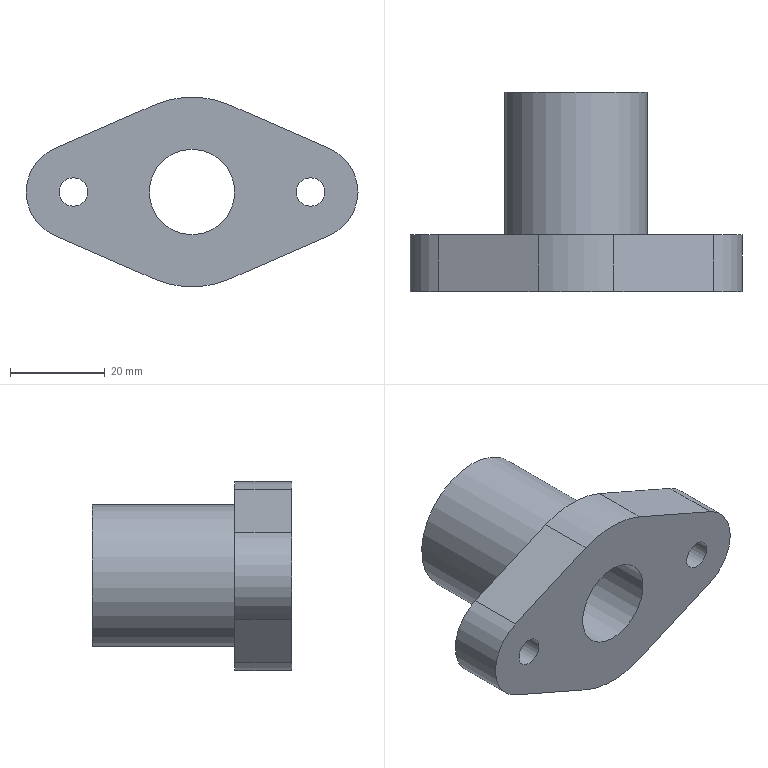Component | NX | GLAND | 1 solid | 15 faces | box 70 x 42 x 40 mm | volume 33070 mm3 | cylinder 8 | plane 7 | commonest cylinder face diameters 40 x2 20 x2 6 x2 30 x1 18 x1
STEP:
#1=CARTESIAN_POINT('',(0.,0.,0.));
#2=DIRECTION('',(0.,0.,1.));
#3=DIRECTION('',(1.,0.,0.));
#4=AXIS2_PLACEMENT_3D('',#1,#2,#3);
#5=CARTESIAN_POINT('',(-29.,-84.,-36.165));
#6=VERTEX_POINT('',#5);
#7=CARTESIAN_POINT('',(-8.,-84.,-45.33));
#8=VERTEX_POINT('',#7);
#9=CARTESIAN_POINT('',(-29.,-84.,-36.165));
#10=DIRECTION('',(0.9165,0.,-0.4));
#11=VECTOR('',#10,1.);
#12=LINE('',#9,#11);
#13=CARTESIAN_POINT('',(-29.,-72.,-36.165));
#14=DIRECTION('',(-0.4,0.,-0.9165));
#15=DIRECTION('',(0.9165,0.,-0.4));
#16=AXIS2_PLACEMENT_3D('',#13,#14,#15);
#17=PLANE('',#16);
#18=CARTESIAN_POINT('',(0.,12.));
#19=DIRECTION('',(1.,0.));
#20=VECTOR('',#19,1.);
#21=LINE('',#18,#20);
#22=(GEOMETRIC_REPRESENTATION_CONTEXT(2)PARAMETRIC_REPRESENTATION_CONTEXT()REPRESENTATION_CONTEXT('',''));
#23=DEFINITIONAL_REPRESENTATION('',(#21),#22);
#24=PCURVE('',#17,#23);
#25=CARTESIAN_POINT('',(0.,-84.,-27.));
#26=DIRECTION('',(0.,-1.,0.));
#27=DIRECTION('',(0.,0.,1.));
#28=AXIS2_PLACEMENT_3D('',#25,#26,#27);
#29=PLANE('',#28);
#30=CARTESIAN_POINT('',(-9.165,29.));
#31=DIRECTION('',(-0.4,-0.9165));
#32=VECTOR('',#31,1.);
#33=LINE('',#30,#32);
#34=(GEOMETRIC_REPRESENTATION_CONTEXT(2)PARAMETRIC_REPRESENTATION_CONTEXT()REPRESENTATION_CONTEXT('',''));
#35=DEFINITIONAL_REPRESENTATION('',(#33),#34);
#36=PCURVE('',#29,#35);
#37=SURFACE_CURVE('',#12,(#24,#36),.PCURVE_S1.);
#38=EDGE_CURVE('',#6,#8,#37,.T.);
#39=ORIENTED_EDGE('',*,*,#38,.F.);
#40=CARTESIAN_POINT('',(-29.,-72.,-36.165));
#41=VERTEX_POINT('',#40);
#42=CARTESIAN_POINT('',(-29.,-72.,-36.165));
#43=DIRECTION('',(0.,-1.,0.));
#44=VECTOR('',#43,1.);
#45=LINE('',#42,#44);
#46=CARTESIAN_POINT('',(0.,0.));
#47=DIRECTION('',(0.,1.));
#48=VECTOR('',#47,1.);
#49=LINE('',#46,#48);
#50=(GEOMETRIC_REPRESENTATION_CONTEXT(2)PARAMETRIC_REPRESENTATION_CONTEXT()REPRESENTATION_CONTEXT('',''));
#51=DEFINITIONAL_REPRESENTATION('',(#49),#50);
#52=PCURVE('',#17,#51);
#53=CARTESIAN_POINT('',(-25.,-72.,-27.));
#54=DIRECTION('',(0.,-1.,0.));
#55=DIRECTION('',(0.,0.,1.));
#56=AXIS2_PLACEMENT_3D('',#53,#54,#55);
#57=CYLINDRICAL_SURFACE('',#56,10.);
#58=CARTESIAN_POINT('',(2.73,0.));
#59=DIRECTION('',(0.,1.));
#60=VECTOR('',#59,1.);
#61=LINE('',#58,#60);
#62=(GEOMETRIC_REPRESENTATION_CONTEXT(2)PARAMETRIC_REPRESENTATION_CONTEXT()REPRESENTATION_CONTEXT('',''));
#63=DEFINITIONAL_REPRESENTATION('',(#61),#62);
#64=PCURVE('',#57,#63);
#65=SURFACE_CURVE('',#45,(#52,#64),.PCURVE_S1.);
#66=EDGE_CURVE('',#41,#6,#65,.T.);
#67=ORIENTED_EDGE('',*,*,#66,.F.);
#68=CARTESIAN_POINT('',(-8.,-72.,-45.33));
#69=VERTEX_POINT('',#68);
#70=CARTESIAN_POINT('',(-29.,-72.,-36.165));
#71=DIRECTION('',(0.9165,0.,-0.4));
#72=VECTOR('',#71,1.);
#73=LINE('',#70,#72);
#74=CARTESIAN_POINT('',(0.,0.));
#75=DIRECTION('',(1.,0.));
#76=VECTOR('',#75,1.);
#77=LINE('',#74,#76);
#78=(GEOMETRIC_REPRESENTATION_CONTEXT(2)PARAMETRIC_REPRESENTATION_CONTEXT()REPRESENTATION_CONTEXT('',''));
#79=DEFINITIONAL_REPRESENTATION('',(#77),#78);
#80=PCURVE('',#17,#79);
#81=CARTESIAN_POINT('',(0.,-72.,-27.));
#82=DIRECTION('',(0.,-1.,0.));
#83=DIRECTION('',(0.,0.,1.));
#84=AXIS2_PLACEMENT_3D('',#81,#82,#83);
#85=PLANE('',#84);
#86=CARTESIAN_POINT('',(-9.165,29.));
#87=DIRECTION('',(-0.4,-0.9165));
#88=VECTOR('',#87,1.);
#89=LINE('',#86,#88);
#90=(GEOMETRIC_REPRESENTATION_CONTEXT(2)PARAMETRIC_REPRESENTATION_CONTEXT()REPRESENTATION_CONTEXT('',''));
#91=DEFINITIONAL_REPRESENTATION('',(#89),#90);
#92=PCURVE('',#85,#91);
#93=SURFACE_CURVE('',#73,(#80,#92),.PCURVE_S1.);
#94=EDGE_CURVE('',#41,#69,#93,.T.);
#95=ORIENTED_EDGE('',*,*,#94,.T.);
#96=CARTESIAN_POINT('',(-8.,-72.,-45.33));
#97=DIRECTION('',(0.,-1.,0.));
#98=VECTOR('',#97,1.);
#99=LINE('',#96,#98);
#100=CARTESIAN_POINT('',(22.913,0.));
#101=DIRECTION('',(0.,1.));
#102=VECTOR('',#101,1.);
#103=LINE('',#100,#102);
#104=(GEOMETRIC_REPRESENTATION_CONTEXT(2)PARAMETRIC_REPRESENTATION_CONTEXT()REPRESENTATION_CONTEXT('',''));
#105=DEFINITIONAL_REPRESENTATION('',(#103),#104);
#106=PCURVE('',#17,#105);
#107=CARTESIAN_POINT('',(0.,-72.,-27.));
#108=DIRECTION('',(0.,-1.,0.));
#109=DIRECTION('',(0.,0.,1.));
#110=AXIS2_PLACEMENT_3D('',#107,#108,#109);
#111=CYLINDRICAL_SURFACE('',#110,20.);
#112=CARTESIAN_POINT('',(2.73,0.));
#113=DIRECTION('',(0.,1.));
#114=VECTOR('',#113,1.);
#115=LINE('',#112,#114);
#116=(GEOMETRIC_REPRESENTATION_CONTEXT(2)PARAMETRIC_REPRESENTATION_CONTEXT()REPRESENTATION_CONTEXT('',''));
#117=DEFINITIONAL_REPRESENTATION('',(#115),#116);
#118=PCURVE('',#111,#117);
#119=SURFACE_CURVE('',#99,(#106,#118),.PCURVE_S1.);
#120=EDGE_CURVE('',#69,#8,#119,.T.);
#121=ORIENTED_EDGE('',*,*,#120,.T.);
#122=EDGE_LOOP('',(#39,#67,#95,#121));
#123=FACE_BOUND('',#122,.T.);
#124=ADVANCED_FACE('',(#123),#17,.T.);
#125=CARTESIAN_POINT('',(8.,-84.,-45.33));
#126=VERTEX_POINT('',#125);
#127=CARTESIAN_POINT('',(0.,-84.,-27.));
#128=DIRECTION('',(0.,-1.,0.));
#129=DIRECTION('',(0.,0.,1.));
#130=AXIS2_PLACEMENT_3D('',#127,#128,#129);
#131=CIRCLE('',#130,20.);
#132=CARTESIAN_POINT('',(0.,12.));
#133=DIRECTION('',(1.,0.));
#134=VECTOR('',#133,1.);
#135=LINE('',#132,#134);
#136=(GEOMETRIC_REPRESENTATION_CONTEXT(2)PARAMETRIC_REPRESENTATION_CONTEXT()REPRESENTATION_CONTEXT('',''));
#137=DEFINITIONAL_REPRESENTATION('',(#135),#136);
#138=PCURVE('',#111,#137);
#139=CARTESIAN_POINT('',(0.,0.));
#140=DIRECTION('',(1.,0.));
#141=AXIS2_PLACEMENT_2D('',#139,#140);
#142=CIRCLE('',#141,20.);
#143=(GEOMETRIC_REPRESENTATION_CONTEXT(2)PARAMETRIC_REPRESENTATION_CONTEXT()REPRESENTATION_CONTEXT('',''));
#144=DEFINITIONAL_REPRESENTATION('',(#142),#143);
#145=PCURVE('',#29,#144);
#146=SURFACE_CURVE('',#131,(#138,#145),.PCURVE_S1.);
#147=EDGE_CURVE('',#8,#126,#146,.T.);
#148=ORIENTED_EDGE('',*,*,#147,.F.);
#149=ORIENTED_EDGE('',*,*,#120,.F.);
#150=CARTESIAN_POINT('',(8.,-72.,-45.33));
#151=VERTEX_POINT('',#150);
#152=CARTESIAN_POINT('',(0.,-72.,-27.));
#153=DIRECTION('',(0.,-1.,0.));
#154=DIRECTION('',(0.,0.,1.));
#155=AXIS2_PLACEMENT_3D('',#152,#153,#154);
#156=CIRCLE('',#155,20.);
#157=CARTESIAN_POINT('',(0.,0.));
#158=DIRECTION('',(1.,0.));
#159=VECTOR('',#158,1.);
#160=LINE('',#157,#159);
#161=(GEOMETRIC_REPRESENTATION_CONTEXT(2)PARAMETRIC_REPRESENTATION_CONTEXT()REPRESENTATION_CONTEXT('',''));
#162=DEFINITIONAL_REPRESENTATION('',(#160),#161);
#163=PCURVE('',#111,#162);
#164=CARTESIAN_POINT('',(0.,0.));
#165=DIRECTION('',(1.,0.));
#166=AXIS2_PLACEMENT_2D('',#164,#165);
#167=CIRCLE('',#166,20.);
#168=(GEOMETRIC_REPRESENTATION_CONTEXT(2)PARAMETRIC_REPRESENTATION_CONTEXT()REPRESENTATION_CONTEXT('',''));
#169=DEFINITIONAL_REPRESENTATION('',(#167),#168);
#170=PCURVE('',#85,#169);
#171=SURFACE_CURVE('',#156,(#163,#170),.PCURVE_S1.);
#172=EDGE_CURVE('',#69,#151,#171,.T.);
#173=ORIENTED_EDGE('',*,*,#172,.T.);
#174=CARTESIAN_POINT('',(8.,-72.,-45.33));
#175=DIRECTION('',(0.,-1.,0.));
#176=VECTOR('',#175,1.);
#177=LINE('',#174,#176);
#178=CARTESIAN_POINT('',(3.553,0.));
#179=DIRECTION('',(0.,1.));
#180=VECTOR('',#179,1.);
#181=LINE('',#178,#180);
#182=(GEOMETRIC_REPRESENTATION_CONTEXT(2)PARAMETRIC_REPRESENTATION_CONTEXT()REPRESENTATION_CONTEXT('',''));
#183=DEFINITIONAL_REPRESENTATION('',(#181),#182);
#184=PCURVE('',#111,#183);
#185=CARTESIAN_POINT('',(8.,-72.,-45.33));
#186=DIRECTION('',(0.4,0.,-0.9165));
#187=DIRECTION('',(0.9165,0.,0.4));
#188=AXIS2_PLACEMENT_3D('',#185,#186,#187);
#189=PLANE('',#188);
#190=CARTESIAN_POINT('',(0.,0.));
#191=DIRECTION('',(0.,1.));
#192=VECTOR('',#191,1.);
#193=LINE('',#190,#192);
#194=(GEOMETRIC_REPRESENTATION_CONTEXT(2)PARAMETRIC_REPRESENTATION_CONTEXT()REPRESENTATION_CONTEXT('',''));
#195=DEFINITIONAL_REPRESENTATION('',(#193),#194);
#196=PCURVE('',#189,#195);
#197=SURFACE_CURVE('',#177,(#184,#196),.PCURVE_S1.);
#198=EDGE_CURVE('',#151,#126,#197,.T.);
#199=ORIENTED_EDGE('',*,*,#198,.T.);
#200=EDGE_LOOP('',(#148,#149,#173,#199));
#201=FACE_BOUND('',#200,.T.);
#202=ADVANCED_FACE('',(#201),#111,.T.);
#203=CARTESIAN_POINT('',(29.,-84.,-36.165));
#204=VERTEX_POINT('',#203);
#205=CARTESIAN_POINT('',(8.,-84.,-45.33));
#206=DIRECTION('',(0.9165,0.,0.4));
#207=VECTOR('',#206,1.);
#208=LINE('',#205,#207);
#209=CARTESIAN_POINT('',(0.,12.));
#210=DIRECTION('',(1.,0.));
#211=VECTOR('',#210,1.);
#212=LINE('',#209,#211);
#213=(GEOMETRIC_REPRESENTATION_CONTEXT(2)PARAMETRIC_REPRESENTATION_CONTEXT()REPRESENTATION_CONTEXT('',''));
#214=DEFINITIONAL_REPRESENTATION('',(#212),#213);
#215=PCURVE('',#189,#214);
#216=CARTESIAN_POINT('',(-18.33,-8.));
#217=DIRECTION('',(0.4,-0.9165));
#218=VECTOR('',#217,1.);
#219=LINE('',#216,#218);
#220=(GEOMETRIC_REPRESENTATION_CONTEXT(2)PARAMETRIC_REPRESENTATION_CONTEXT()REPRESENTATION_CONTEXT('',''));
#221=DEFINITIONAL_REPRESENTATION('',(#219),#220);
#222=PCURVE('',#29,#221);
#223=SURFACE_CURVE('',#208,(#215,#222),.PCURVE_S1.);
#224=EDGE_CURVE('',#126,#204,#223,.T.);
#225=ORIENTED_EDGE('',*,*,#224,.F.);
#226=ORIENTED_EDGE('',*,*,#198,.F.);
#227=CARTESIAN_POINT('',(29.,-72.,-36.165));
#228=VERTEX_POINT('',#227);
#229=CARTESIAN_POINT('',(8.,-72.,-45.33));
#230=DIRECTION('',(0.9165,0.,0.4));
#231=VECTOR('',#230,1.);
#232=LINE('',#229,#231);
#233=CARTESIAN_POINT('',(0.,0.));
#234=DIRECTION('',(1.,0.));
#235=VECTOR('',#234,1.);
#236=LINE('',#233,#235);
#237=(GEOMETRIC_REPRESENTATION_CONTEXT(2)PARAMETRIC_REPRESENTATION_CONTEXT()REPRESENTATION_CONTEXT('',''));
#238=DEFINITIONAL_REPRESENTATION('',(#236),#237);
#239=PCURVE('',#189,#238);
#240=CARTESIAN_POINT('',(-18.33,-8.));
#241=DIRECTION('',(0.4,-0.9165));
#242=VECTOR('',#241,1.);
#243=LINE('',#240,#242);
#244=(GEOMETRIC_REPRESENTATION_CONTEXT(2)PARAMETRIC_REPRESENTATION_CONTEXT()REPRESENTATION_CONTEXT('',''));
#245=DEFINITIONAL_REPRESENTATION('',(#243),#244);
#246=PCURVE('',#85,#245);
#247=SURFACE_CURVE('',#232,(#239,#246),.PCURVE_S1.);
#248=EDGE_CURVE('',#151,#228,#247,.T.);
#249=ORIENTED_EDGE('',*,*,#248,.T.);
#250=CARTESIAN_POINT('',(29.,-72.,-36.165));
#251=DIRECTION('',(0.,-1.,0.));
#252=VECTOR('',#251,1.);
#253=LINE('',#250,#252);
#254=CARTESIAN_POINT('',(22.913,0.));
#255=DIRECTION('',(0.,1.));
#256=VECTOR('',#255,1.);
#257=LINE('',#254,#256);
#258=(GEOMETRIC_REPRESENTATION_CONTEXT(2)PARAMETRIC_REPRESENTATION_CONTEXT()REPRESENTATION_CONTEXT('',''));
#259=DEFINITIONAL_REPRESENTATION('',(#257),#258);
#260=PCURVE('',#189,#259);
#261=CARTESIAN_POINT('',(25.,-72.,-27.));
#262=DIRECTION('',(0.,-1.,0.));
#263=DIRECTION('',(0.,0.,1.));
#264=AXIS2_PLACEMENT_3D('',#261,#262,#263);
#265=CYLINDRICAL_SURFACE('',#264,10.);
#266=CARTESIAN_POINT('',(3.553,0.));
#267=DIRECTION('',(0.,1.));
#268=VECTOR('',#267,1.);
#269=LINE('',#266,#268);
#270=(GEOMETRIC_REPRESENTATION_CONTEXT(2)PARAMETRIC_REPRESENTATION_CONTEXT()REPRESENTATION_CONTEXT('',''));
#271=DEFINITIONAL_REPRESENTATION('',(#269),#270);
#272=PCURVE('',#265,#271);
#273=SURFACE_CURVE('',#253,(#260,#272),.PCURVE_S1.);
#274=EDGE_CURVE('',#228,#204,#273,.T.);
#275=ORIENTED_EDGE('',*,*,#274,.T.);
#276=EDGE_LOOP('',(#225,#226,#249,#275));
#277=FACE_BOUND('',#276,.T.);
#278=ADVANCED_FACE('',(#277),#189,.T.);
#279=CARTESIAN_POINT('',(29.,-84.,-17.835));
#280=VERTEX_POINT('',#279);
#281=CARTESIAN_POINT('',(25.,-84.,-27.));
#282=DIRECTION('',(0.,-1.,0.));
#283=DIRECTION('',(0.,0.,1.));
#284=AXIS2_PLACEMENT_3D('',#281,#282,#283);
#285=CIRCLE('',#284,10.);
#286=CARTESIAN_POINT('',(-0.,12.));
#287=DIRECTION('',(1.,0.));
#288=VECTOR('',#287,1.);
#289=LINE('',#286,#288);
#290=(GEOMETRIC_REPRESENTATION_CONTEXT(2)PARAMETRIC_REPRESENTATION_CONTEXT()REPRESENTATION_CONTEXT('',''));
#291=DEFINITIONAL_REPRESENTATION('',(#289),#290);
#292=PCURVE('',#265,#291);
#293=CARTESIAN_POINT('',(0.,-25.));
#294=DIRECTION('',(1.,0.));
#295=AXIS2_PLACEMENT_2D('',#293,#294);
#296=CIRCLE('',#295,10.);
#297=(GEOMETRIC_REPRESENTATION_CONTEXT(2)PARAMETRIC_REPRESENTATION_CONTEXT()REPRESENTATION_CONTEXT('',''));
#298=DEFINITIONAL_REPRESENTATION('',(#296),#297);
#299=PCURVE('',#29,#298);
#300=SURFACE_CURVE('',#285,(#292,#299),.PCURVE_S1.);
#301=EDGE_CURVE('',#204,#280,#300,.T.);
#302=ORIENTED_EDGE('',*,*,#301,.F.);
#303=ORIENTED_EDGE('',*,*,#274,.F.);
#304=CARTESIAN_POINT('',(29.,-72.,-17.835));
#305=VERTEX_POINT('',#304);
#306=CARTESIAN_POINT('',(25.,-72.,-27.));
#307=DIRECTION('',(0.,-1.,0.));
#308=DIRECTION('',(0.,0.,1.));
#309=AXIS2_PLACEMENT_3D('',#306,#307,#308);
#310=CIRCLE('',#309,10.);
#311=CARTESIAN_POINT('',(-0.,0.));
#312=DIRECTION('',(1.,0.));
#313=VECTOR('',#312,1.);
#314=LINE('',#311,#313);
#315=(GEOMETRIC_REPRESENTATION_CONTEXT(2)PARAMETRIC_REPRESENTATION_CONTEXT()REPRESENTATION_CONTEXT('',''));
#316=DEFINITIONAL_REPRESENTATION('',(#314),#315);
#317=PCURVE('',#265,#316);
#318=CARTESIAN_POINT('',(0.,-25.));
#319=DIRECTION('',(1.,0.));
#320=AXIS2_PLACEMENT_2D('',#318,#319);
#321=CIRCLE('',#320,10.);
#322=(GEOMETRIC_REPRESENTATION_CONTEXT(2)PARAMETRIC_REPRESENTATION_CONTEXT()REPRESENTATION_CONTEXT('',''));
#323=DEFINITIONAL_REPRESENTATION('',(#321),#322);
#324=PCURVE('',#85,#323);
#325=SURFACE_CURVE('',#310,(#317,#324),.PCURVE_S1.);
#326=EDGE_CURVE('',#228,#305,#325,.T.);
#327=ORIENTED_EDGE('',*,*,#326,.T.);
#328=CARTESIAN_POINT('',(29.,-72.,-17.835));
#329=DIRECTION('',(0.,-1.,0.));
#330=VECTOR('',#329,1.);
#331=LINE('',#328,#330);
#332=CARTESIAN_POINT('',(5.872,0.));
#333=DIRECTION('',(0.,1.));
#334=VECTOR('',#333,1.);
#335=LINE('',#332,#334);
#336=(GEOMETRIC_REPRESENTATION_CONTEXT(2)PARAMETRIC_REPRESENTATION_CONTEXT()REPRESENTATION_CONTEXT('',''));
#337=DEFINITIONAL_REPRESENTATION('',(#335),#336);
#338=PCURVE('',#265,#337);
#339=CARTESIAN_POINT('',(29.,-72.,-17.835));
#340=DIRECTION('',(0.4,0.,0.9165));
#341=DIRECTION('',(-0.9165,0.,0.4));
#342=AXIS2_PLACEMENT_3D('',#339,#340,#341);
#343=PLANE('',#342);
#344=CARTESIAN_POINT('',(-0.,0.));
#345=DIRECTION('',(0.,1.));
#346=VECTOR('',#345,1.);
#347=LINE('',#344,#346);
#348=(GEOMETRIC_REPRESENTATION_CONTEXT(2)PARAMETRIC_REPRESENTATION_CONTEXT()REPRESENTATION_CONTEXT('',''));
#349=DEFINITIONAL_REPRESENTATION('',(#347),#348);
#350=PCURVE('',#343,#349);
#351=SURFACE_CURVE('',#331,(#338,#350),.PCURVE_S1.);
#352=EDGE_CURVE('',#305,#280,#351,.T.);
#353=ORIENTED_EDGE('',*,*,#352,.T.);
#354=EDGE_LOOP('',(#302,#303,#327,#353));
#355=FACE_BOUND('',#354,.T.);
#356=ADVANCED_FACE('',(#355),#265,.T.);
#357=CARTESIAN_POINT('',(8.,-84.,-8.67));
#358=VERTEX_POINT('',#357);
#359=CARTESIAN_POINT('',(29.,-84.,-17.835));
#360=DIRECTION('',(-0.9165,0.,0.4));
#361=VECTOR('',#360,1.);
#362=LINE('',#359,#361);
#363=CARTESIAN_POINT('',(0.,12.));
#364=DIRECTION('',(1.,0.));
#365=VECTOR('',#364,1.);
#366=LINE('',#363,#365);
#367=(GEOMETRIC_REPRESENTATION_CONTEXT(2)PARAMETRIC_REPRESENTATION_CONTEXT()REPRESENTATION_CONTEXT('',''));
#368=DEFINITIONAL_REPRESENTATION('',(#366),#367);
#369=PCURVE('',#343,#368);
#370=CARTESIAN_POINT('',(9.165,-29.));
#371=DIRECTION('',(0.4,0.9165));
#372=VECTOR('',#371,1.);
#373=LINE('',#370,#372);
#374=(GEOMETRIC_REPRESENTATION_CONTEXT(2)PARAMETRIC_REPRESENTATION_CONTEXT()REPRESENTATION_CONTEXT('',''));
#375=DEFINITIONAL_REPRESENTATION('',(#373),#374);
#376=PCURVE('',#29,#375);
#377=SURFACE_CURVE('',#362,(#369,#376),.PCURVE_S1.);
#378=EDGE_CURVE('',#280,#358,#377,.T.);
#379=ORIENTED_EDGE('',*,*,#378,.F.);
#380=ORIENTED_EDGE('',*,*,#352,.F.);
#381=CARTESIAN_POINT('',(8.,-72.,-8.67));
#382=VERTEX_POINT('',#381);
#383=CARTESIAN_POINT('',(29.,-72.,-17.835));
#384=DIRECTION('',(-0.9165,0.,0.4));
#385=VECTOR('',#384,1.);
#386=LINE('',#383,#385);
#387=CARTESIAN_POINT('',(0.,0.));
#388=DIRECTION('',(1.,0.));
#389=VECTOR('',#388,1.);
#390=LINE('',#387,#389);
#391=(GEOMETRIC_REPRESENTATION_CONTEXT(2)PARAMETRIC_REPRESENTATION_CONTEXT()REPRESENTATION_CONTEXT('',''));
#392=DEFINITIONAL_REPRESENTATION('',(#390),#391);
#393=PCURVE('',#343,#392);
#394=CARTESIAN_POINT('',(9.165,-29.));
#395=DIRECTION('',(0.4,0.9165));
#396=VECTOR('',#395,1.);
#397=LINE('',#394,#396);
#398=(GEOMETRIC_REPRESENTATION_CONTEXT(2)PARAMETRIC_REPRESENTATION_CONTEXT()REPRESENTATION_CONTEXT('',''));
#399=DEFINITIONAL_REPRESENTATION('',(#397),#398);
#400=PCURVE('',#85,#399);
#401=SURFACE_CURVE('',#386,(#393,#400),.PCURVE_S1.);
#402=EDGE_CURVE('',#305,#382,#401,.T.);
#403=ORIENTED_EDGE('',*,*,#402,.T.);
#404=CARTESIAN_POINT('',(8.,-72.,-8.67));
#405=DIRECTION('',(0.,-1.,0.));
#406=VECTOR('',#405,1.);
#407=LINE('',#404,#406);
#408=CARTESIAN_POINT('',(22.913,0.));
#409=DIRECTION('',(0.,1.));
#410=VECTOR('',#409,1.);
#411=LINE('',#408,#410);
#412=(GEOMETRIC_REPRESENTATION_CONTEXT(2)PARAMETRIC_REPRESENTATION_CONTEXT()REPRESENTATION_CONTEXT('',''));
#413=DEFINITIONAL_REPRESENTATION('',(#411),#412);
#414=PCURVE('',#343,#413);
#415=CARTESIAN_POINT('',(0.,-72.,-27.));
#416=DIRECTION('',(0.,-1.,0.));
#417=DIRECTION('',(0.,0.,1.));
#418=AXIS2_PLACEMENT_3D('',#415,#416,#417);
#419=CYLINDRICAL_SURFACE('',#418,20.);
#420=CARTESIAN_POINT('',(5.872,0.));
#421=DIRECTION('',(0.,1.));
#422=VECTOR('',#421,1.);
#423=LINE('',#420,#422);
#424=(GEOMETRIC_REPRESENTATION_CONTEXT(2)PARAMETRIC_REPRESENTATION_CONTEXT()REPRESENTATION_CONTEXT('',''));
#425=DEFINITIONAL_REPRESENTATION('',(#423),#424);
#426=PCURVE('',#419,#425);
#427=SURFACE_CURVE('',#407,(#414,#426),.PCURVE_S1.);
#428=EDGE_CURVE('',#382,#358,#427,.T.);
#429=ORIENTED_EDGE('',*,*,#428,.T.);
#430=EDGE_LOOP('',(#379,#380,#403,#429));
#431=FACE_BOUND('',#430,.T.);
#432=ADVANCED_FACE('',(#431),#343,.T.);
#433=CARTESIAN_POINT('',(-8.,-84.,-8.67));
#434=VERTEX_POINT('',#433);
#435=CARTESIAN_POINT('',(0.,-84.,-27.));
#436=DIRECTION('',(0.,-1.,0.));
#437=DIRECTION('',(0.,0.,1.));
#438=AXIS2_PLACEMENT_3D('',#435,#436,#437);
#439=CIRCLE('',#438,20.);
#440=CARTESIAN_POINT('',(0.,12.));
#441=DIRECTION('',(1.,0.));
#442=VECTOR('',#441,1.);
#443=LINE('',#440,#442);
#444=(GEOMETRIC_REPRESENTATION_CONTEXT(2)PARAMETRIC_REPRESENTATION_CONTEXT()REPRESENTATION_CONTEXT('',''));
#445=DEFINITIONAL_REPRESENTATION('',(#443),#444);
#446=PCURVE('',#419,#445);
#447=CARTESIAN_POINT('',(0.,0.));
#448=DIRECTION('',(1.,0.));
#449=AXIS2_PLACEMENT_2D('',#447,#448);
#450=CIRCLE('',#449,20.);
#451=(GEOMETRIC_REPRESENTATION_CONTEXT(2)PARAMETRIC_REPRESENTATION_CONTEXT()REPRESENTATION_CONTEXT('',''));
#452=DEFINITIONAL_REPRESENTATION('',(#450),#451);
#453=PCURVE('',#29,#452);
#454=SURFACE_CURVE('',#439,(#446,#453),.PCURVE_S1.);
#455=EDGE_CURVE('',#358,#434,#454,.T.);
#456=ORIENTED_EDGE('',*,*,#455,.F.);
#457=ORIENTED_EDGE('',*,*,#428,.F.);
#458=CARTESIAN_POINT('',(-8.,-72.,-8.67));
#459=VERTEX_POINT('',#458);
#460=CARTESIAN_POINT('',(0.,-72.,-27.));
#461=DIRECTION('',(0.,-1.,0.));
#462=DIRECTION('',(0.,0.,1.));
#463=AXIS2_PLACEMENT_3D('',#460,#461,#462);
#464=CIRCLE('',#463,20.);
#465=CARTESIAN_POINT('',(0.,0.));
#466=DIRECTION('',(1.,0.));
#467=VECTOR('',#466,1.);
#468=LINE('',#465,#467);
#469=(GEOMETRIC_REPRESENTATION_CONTEXT(2)PARAMETRIC_REPRESENTATION_CONTEXT()REPRESENTATION_CONTEXT('',''));
#470=DEFINITIONAL_REPRESENTATION('',(#468),#469);
#471=PCURVE('',#419,#470);
#472=CARTESIAN_POINT('',(0.,0.));
#473=DIRECTION('',(1.,0.));
#474=AXIS2_PLACEMENT_2D('',#472,#473);
#475=CIRCLE('',#474,20.);
#476=(GEOMETRIC_REPRESENTATION_CONTEXT(2)PARAMETRIC_REPRESENTATION_CONTEXT()REPRESENTATION_CONTEXT('',''));
#477=DEFINITIONAL_REPRESENTATION('',(#475),#476);
#478=PCURVE('',#85,#477);
#479=SURFACE_CURVE('',#464,(#471,#478),.PCURVE_S1.);
#480=EDGE_CURVE('',#382,#459,#479,.T.);
#481=ORIENTED_EDGE('',*,*,#480,.T.);
#482=CARTESIAN_POINT('',(-8.,-72.,-8.67));
#483=DIRECTION('',(0.,-1.,0.));
#484=VECTOR('',#483,1.);
#485=LINE('',#482,#484);
#486=CARTESIAN_POINT('',(6.695,0.));
#487=DIRECTION('',(0.,1.));
#488=VECTOR('',#487,1.);
#489=LINE('',#486,#488);
#490=(GEOMETRIC_REPRESENTATION_CONTEXT(2)PARAMETRIC_REPRESENTATION_CONTEXT()REPRESENTATION_CONTEXT('',''));
#491=DEFINITIONAL_REPRESENTATION('',(#489),#490);
#492=PCURVE('',#419,#491);
#493=CARTESIAN_POINT('',(-8.,-72.,-8.67));
#494=DIRECTION('',(-0.4,0.,0.9165));
#495=DIRECTION('',(-0.9165,0.,-0.4));
#496=AXIS2_PLACEMENT_3D('',#493,#494,#495);
#497=PLANE('',#496);
#498=CARTESIAN_POINT('',(-0.,0.));
#499=DIRECTION('',(0.,1.));
#500=VECTOR('',#499,1.);
#501=LINE('',#498,#500);
#502=(GEOMETRIC_REPRESENTATION_CONTEXT(2)PARAMETRIC_REPRESENTATION_CONTEXT()REPRESENTATION_CONTEXT('',''));
#503=DEFINITIONAL_REPRESENTATION('',(#501),#502);
#504=PCURVE('',#497,#503);
#505=SURFACE_CURVE('',#485,(#492,#504),.PCURVE_S1.);
#506=EDGE_CURVE('',#459,#434,#505,.T.);
#507=ORIENTED_EDGE('',*,*,#506,.T.);
#508=EDGE_LOOP('',(#456,#457,#481,#507));
#509=FACE_BOUND('',#508,.T.);
#510=ADVANCED_FACE('',(#509),#419,.T.);
#511=CARTESIAN_POINT('',(-29.,-84.,-17.835));
#512=VERTEX_POINT('',#511);
#513=CARTESIAN_POINT('',(-8.,-84.,-8.67));
#514=DIRECTION('',(-0.9165,0.,-0.4));
#515=VECTOR('',#514,1.);
#516=LINE('',#513,#515);
#517=CARTESIAN_POINT('',(0.,12.));
#518=DIRECTION('',(1.,0.));
#519=VECTOR('',#518,1.);
#520=LINE('',#517,#519);
#521=(GEOMETRIC_REPRESENTATION_CONTEXT(2)PARAMETRIC_REPRESENTATION_CONTEXT()REPRESENTATION_CONTEXT('',''));
#522=DEFINITIONAL_REPRESENTATION('',(#520),#521);
#523=PCURVE('',#497,#522);
#524=CARTESIAN_POINT('',(18.33,8.));
#525=DIRECTION('',(-0.4,0.9165));
#526=VECTOR('',#525,1.);
#527=LINE('',#524,#526);
#528=(GEOMETRIC_REPRESENTATION_CONTEXT(2)PARAMETRIC_REPRESENTATION_CONTEXT()REPRESENTATION_CONTEXT('',''));
#529=DEFINITIONAL_REPRESENTATION('',(#527),#528);
#530=PCURVE('',#29,#529);
#531=SURFACE_CURVE('',#516,(#523,#530),.PCURVE_S1.);
#532=EDGE_CURVE('',#434,#512,#531,.T.);
#533=ORIENTED_EDGE('',*,*,#532,.F.);
#534=ORIENTED_EDGE('',*,*,#506,.F.);
#535=CARTESIAN_POINT('',(-29.,-72.,-17.835));
#536=VERTEX_POINT('',#535);
#537=CARTESIAN_POINT('',(-8.,-72.,-8.67));
#538=DIRECTION('',(-0.9165,0.,-0.4));
#539=VECTOR('',#538,1.);
#540=LINE('',#537,#539);
#541=CARTESIAN_POINT('',(0.,0.));
#542=DIRECTION('',(1.,0.));
#543=VECTOR('',#542,1.);
#544=LINE('',#541,#543);
#545=(GEOMETRIC_REPRESENTATION_CONTEXT(2)PARAMETRIC_REPRESENTATION_CONTEXT()REPRESENTATION_CONTEXT('',''));
#546=DEFINITIONAL_REPRESENTATION('',(#544),#545);
#547=PCURVE('',#497,#546);
#548=CARTESIAN_POINT('',(18.33,8.));
#549=DIRECTION('',(-0.4,0.9165));
#550=VECTOR('',#549,1.);
#551=LINE('',#548,#550);
#552=(GEOMETRIC_REPRESENTATION_CONTEXT(2)PARAMETRIC_REPRESENTATION_CONTEXT()REPRESENTATION_CONTEXT('',''));
#553=DEFINITIONAL_REPRESENTATION('',(#551),#552);
#554=PCURVE('',#85,#553);
#555=SURFACE_CURVE('',#540,(#547,#554),.PCURVE_S1.);
#556=EDGE_CURVE('',#459,#536,#555,.T.);
#557=ORIENTED_EDGE('',*,*,#556,.T.);
#558=CARTESIAN_POINT('',(-29.,-72.,-17.835));
#559=DIRECTION('',(0.,-1.,0.));
#560=VECTOR('',#559,1.);
#561=LINE('',#558,#560);
#562=CARTESIAN_POINT('',(22.913,0.));
#563=DIRECTION('',(0.,1.));
#564=VECTOR('',#563,1.);
#565=LINE('',#562,#564);
#566=(GEOMETRIC_REPRESENTATION_CONTEXT(2)PARAMETRIC_REPRESENTATION_CONTEXT()REPRESENTATION_CONTEXT('',''));
#567=DEFINITIONAL_REPRESENTATION('',(#565),#566);
#568=PCURVE('',#497,#567);
#569=CARTESIAN_POINT('',(0.4115,0.));
#570=DIRECTION('',(0.,1.));
#571=VECTOR('',#570,1.);
#572=LINE('',#569,#571);
#573=(GEOMETRIC_REPRESENTATION_CONTEXT(2)PARAMETRIC_REPRESENTATION_CONTEXT()REPRESENTATION_CONTEXT('',''));
#574=DEFINITIONAL_REPRESENTATION('',(#572),#573);
#575=PCURVE('',#57,#574);
#576=SURFACE_CURVE('',#561,(#568,#575),.PCURVE_S1.);
#577=EDGE_CURVE('',#536,#512,#576,.T.);
#578=ORIENTED_EDGE('',*,*,#577,.T.);
#579=EDGE_LOOP('',(#533,#534,#557,#578));
#580=FACE_BOUND('',#579,.T.);
#581=ADVANCED_FACE('',(#580),#497,.T.);
#582=CARTESIAN_POINT('',(-25.,-84.,-27.));
#583=DIRECTION('',(0.,-1.,0.));
#584=DIRECTION('',(0.,0.,1.));
#585=AXIS2_PLACEMENT_3D('',#582,#583,#584);
#586=CIRCLE('',#585,10.);
#587=CARTESIAN_POINT('',(-0.,12.));
#588=DIRECTION('',(1.,0.));
#589=VECTOR('',#588,1.);
#590=LINE('',#587,#589);
#591=(GEOMETRIC_REPRESENTATION_CONTEXT(2)PARAMETRIC_REPRESENTATION_CONTEXT()REPRESENTATION_CONTEXT('',''));
#592=DEFINITIONAL_REPRESENTATION('',(#590),#591);
#593=PCURVE('',#57,#592);
#594=CARTESIAN_POINT('',(0.,25.));
#595=DIRECTION('',(1.,0.));
#596=AXIS2_PLACEMENT_2D('',#594,#595);
#597=CIRCLE('',#596,10.);
#598=(GEOMETRIC_REPRESENTATION_CONTEXT(2)PARAMETRIC_REPRESENTATION_CONTEXT()REPRESENTATION_CONTEXT('',''));
#599=DEFINITIONAL_REPRESENTATION('',(#597),#598);
#600=PCURVE('',#29,#599);
#601=SURFACE_CURVE('',#586,(#593,#600),.PCURVE_S1.);
#602=EDGE_CURVE('',#512,#6,#601,.T.);
#603=ORIENTED_EDGE('',*,*,#602,.F.);
#604=ORIENTED_EDGE('',*,*,#577,.F.);
#605=CARTESIAN_POINT('',(-25.,-72.,-27.));
#606=DIRECTION('',(0.,-1.,0.));
#607=DIRECTION('',(0.,0.,1.));
#608=AXIS2_PLACEMENT_3D('',#605,#606,#607);
#609=CIRCLE('',#608,10.);
#610=CARTESIAN_POINT('',(-0.,0.));
#611=DIRECTION('',(1.,0.));
#612=VECTOR('',#611,1.);
#613=LINE('',#610,#612);
#614=(GEOMETRIC_REPRESENTATION_CONTEXT(2)PARAMETRIC_REPRESENTATION_CONTEXT()REPRESENTATION_CONTEXT('',''));
#615=DEFINITIONAL_REPRESENTATION('',(#613),#614);
#616=PCURVE('',#57,#615);
#617=CARTESIAN_POINT('',(0.,25.));
#618=DIRECTION('',(1.,0.));
#619=AXIS2_PLACEMENT_2D('',#617,#618);
#620=CIRCLE('',#619,10.);
#621=(GEOMETRIC_REPRESENTATION_CONTEXT(2)PARAMETRIC_REPRESENTATION_CONTEXT()REPRESENTATION_CONTEXT('',''));
#622=DEFINITIONAL_REPRESENTATION('',(#620),#621);
#623=PCURVE('',#85,#622);
#624=SURFACE_CURVE('',#609,(#616,#623),.PCURVE_S1.);
#625=EDGE_CURVE('',#536,#41,#624,.T.);
#626=ORIENTED_EDGE('',*,*,#625,.T.);
#627=ORIENTED_EDGE('',*,*,#66,.T.);
#628=EDGE_LOOP('',(#603,#604,#626,#627));
#629=FACE_BOUND('',#628,.T.);
#630=ADVANCED_FACE('',(#629),#57,.T.);
#631=CARTESIAN_POINT('',(0.,-72.,-12.));
#632=VERTEX_POINT('',#631);
#633=CARTESIAN_POINT('',(0.,-72.,-27.));
#634=DIRECTION('',(0.,1.,0.));
#635=DIRECTION('',(0.,0.,1.));
#636=AXIS2_PLACEMENT_3D('',#633,#634,#635);
#637=CIRCLE('',#636,15.);
#638=CARTESIAN_POINT('',(15.,0.));
#639=CARTESIAN_POINT('',(15.,-25.981));
#640=CARTESIAN_POINT('',(-7.5,-12.99));
#641=CARTESIAN_POINT('',(-30.,-0.));
#642=CARTESIAN_POINT('',(-7.5,12.99));
#643=CARTESIAN_POINT('',(15.,25.981));
#644=CARTESIAN_POINT('',(15.,0.));
#645=(BOUNDED_CURVE()B_SPLINE_CURVE(2,(#638,#639,#640,#641,#642,#643,#644),.UNSPECIFIED.,.T.,.F.)B_SPLINE_CURVE_WITH_KNOTS((1,2,2,2,2,1),(-2.094,0.,2.094,4.189,6.283,8.378),.UNSPECIFIED.)CURVE()GEOMETRIC_REPRESENTATION_ITEM()RATIONAL_B_SPLINE_CURVE((1.,0.5,1.,0.5,1.,0.5,1.))REPRESENTATION_ITEM(''));
#646=(GEOMETRIC_REPRESENTATION_CONTEXT(2)PARAMETRIC_REPRESENTATION_CONTEXT()REPRESENTATION_CONTEXT('',''));
#647=DEFINITIONAL_REPRESENTATION('',(#645),#646);
#648=PCURVE('',#85,#647);
#649=CARTESIAN_POINT('',(0.,-72.,-27.));
#650=DIRECTION('',(0.,1.,0.));
#651=DIRECTION('',(0.,0.,1.));
#652=AXIS2_PLACEMENT_3D('',#649,#650,#651);
#653=CYLINDRICAL_SURFACE('',#652,15.);
#654=CARTESIAN_POINT('',(0.,0.));
#655=DIRECTION('',(1.,0.));
#656=VECTOR('',#655,1.);
#657=LINE('',#654,#656);
#658=(GEOMETRIC_REPRESENTATION_CONTEXT(2)PARAMETRIC_REPRESENTATION_CONTEXT()REPRESENTATION_CONTEXT('',''));
#659=DEFINITIONAL_REPRESENTATION('',(#657),#658);
#660=PCURVE('',#653,#659);
#661=SURFACE_CURVE('',#637,(#648,#660),.PCURVE_S1.);
#662=EDGE_CURVE('',#632,#632,#661,.T.);
#663=ORIENTED_EDGE('',*,*,#662,.F.);
#664=EDGE_LOOP('',(#663));
#665=FACE_BOUND('',#664,.T.);
#666=CARTESIAN_POINT('',(-25.,-72.,-24.));
#667=VERTEX_POINT('',#666);
#668=CARTESIAN_POINT('',(-25.,-72.,-27.));
#669=DIRECTION('',(0.,-1.,0.));
#670=DIRECTION('',(0.,0.,1.));
#671=AXIS2_PLACEMENT_3D('',#668,#669,#670);
#672=CIRCLE('',#671,3.);
#673=CARTESIAN_POINT('',(0.,25.));
#674=DIRECTION('',(1.,0.));
#675=AXIS2_PLACEMENT_2D('',#673,#674);
#676=CIRCLE('',#675,3.);
#677=(GEOMETRIC_REPRESENTATION_CONTEXT(2)PARAMETRIC_REPRESENTATION_CONTEXT()REPRESENTATION_CONTEXT('',''));
#678=DEFINITIONAL_REPRESENTATION('',(#676),#677);
#679=PCURVE('',#85,#678);
#680=CARTESIAN_POINT('',(-25.,-72.,-27.));
#681=DIRECTION('',(0.,-1.,0.));
#682=DIRECTION('',(0.,0.,1.));
#683=AXIS2_PLACEMENT_3D('',#680,#681,#682);
#684=CYLINDRICAL_SURFACE('',#683,3.);
#685=CARTESIAN_POINT('',(0.,0.));
#686=DIRECTION('',(1.,0.));
#687=VECTOR('',#686,1.);
#688=LINE('',#685,#687);
#689=(GEOMETRIC_REPRESENTATION_CONTEXT(2)PARAMETRIC_REPRESENTATION_CONTEXT()REPRESENTATION_CONTEXT('',''));
#690=DEFINITIONAL_REPRESENTATION('',(#688),#689);
#691=PCURVE('',#684,#690);
#692=SURFACE_CURVE('',#672,(#679,#691),.PCURVE_S1.);
#693=EDGE_CURVE('',#667,#667,#692,.T.);
#694=ORIENTED_EDGE('',*,*,#693,.T.);
#695=EDGE_LOOP('',(#694));
#696=FACE_BOUND('',#695,.T.);
#697=CARTESIAN_POINT('',(25.,-72.,-24.));
#698=VERTEX_POINT('',#697);
#699=CARTESIAN_POINT('',(25.,-72.,-27.));
#700=DIRECTION('',(0.,-1.,0.));
#701=DIRECTION('',(0.,0.,1.));
#702=AXIS2_PLACEMENT_3D('',#699,#700,#701);
#703=CIRCLE('',#702,3.);
#704=CARTESIAN_POINT('',(0.,-25.));
#705=DIRECTION('',(1.,0.));
#706=AXIS2_PLACEMENT_2D('',#704,#705);
#707=CIRCLE('',#706,3.);
#708=(GEOMETRIC_REPRESENTATION_CONTEXT(2)PARAMETRIC_REPRESENTATION_CONTEXT()REPRESENTATION_CONTEXT('',''));
#709=DEFINITIONAL_REPRESENTATION('',(#707),#708);
#710=PCURVE('',#85,#709);
#711=CARTESIAN_POINT('',(25.,-72.,-27.));
#712=DIRECTION('',(0.,-1.,0.));
#713=DIRECTION('',(0.,0.,1.));
#714=AXIS2_PLACEMENT_3D('',#711,#712,#713);
#715=CYLINDRICAL_SURFACE('',#714,3.);
#716=CARTESIAN_POINT('',(0.,0.));
#717=DIRECTION('',(1.,0.));
#718=VECTOR('',#717,1.);
#719=LINE('',#716,#718);
#720=(GEOMETRIC_REPRESENTATION_CONTEXT(2)PARAMETRIC_REPRESENTATION_CONTEXT()REPRESENTATION_CONTEXT('',''));
#721=DEFINITIONAL_REPRESENTATION('',(#719),#720);
#722=PCURVE('',#715,#721);
#723=SURFACE_CURVE('',#703,(#710,#722),.PCURVE_S1.);
#724=EDGE_CURVE('',#698,#698,#723,.T.);
#725=ORIENTED_EDGE('',*,*,#724,.T.);
#726=EDGE_LOOP('',(#725));
#727=FACE_BOUND('',#726,.T.);
#728=ORIENTED_EDGE('',*,*,#94,.F.);
#729=ORIENTED_EDGE('',*,*,#625,.F.);
#730=ORIENTED_EDGE('',*,*,#556,.F.);
#731=ORIENTED_EDGE('',*,*,#480,.F.);
#732=ORIENTED_EDGE('',*,*,#402,.F.);
#733=ORIENTED_EDGE('',*,*,#326,.F.);
#734=ORIENTED_EDGE('',*,*,#248,.F.);
#735=ORIENTED_EDGE('',*,*,#172,.F.);
#736=EDGE_LOOP('',(#728,#729,#730,#731,#732,#733,#734,#735));
#737=FACE_BOUND('',#736,.T.);
#738=ADVANCED_FACE('',(#665,#696,#727,#737),#85,.F.);
#739=CARTESIAN_POINT('',(0.,-84.,-18.));
#740=VERTEX_POINT('',#739);
#741=CARTESIAN_POINT('',(0.,-84.,-27.));
#742=DIRECTION('',(0.,-1.,0.));
#743=DIRECTION('',(0.,0.,1.));
#744=AXIS2_PLACEMENT_3D('',#741,#742,#743);
#745=CIRCLE('',#744,9.);
#746=CARTESIAN_POINT('',(0.,0.));
#747=DIRECTION('',(1.,0.));
#748=AXIS2_PLACEMENT_2D('',#746,#747);
#749=CIRCLE('',#748,9.);
#750=(GEOMETRIC_REPRESENTATION_CONTEXT(2)PARAMETRIC_REPRESENTATION_CONTEXT()REPRESENTATION_CONTEXT('',''));
#751=DEFINITIONAL_REPRESENTATION('',(#749),#750);
#752=PCURVE('',#29,#751);
#753=CARTESIAN_POINT('',(0.,-42.,-27.));
#754=DIRECTION('',(0.,-1.,0.));
#755=DIRECTION('',(0.,0.,1.));
#756=AXIS2_PLACEMENT_3D('',#753,#754,#755);
#757=CYLINDRICAL_SURFACE('',#756,9.);
#758=CARTESIAN_POINT('',(0.,42.));
#759=DIRECTION('',(1.,0.));
#760=VECTOR('',#759,1.);
#761=LINE('',#758,#760);
#762=(GEOMETRIC_REPRESENTATION_CONTEXT(2)PARAMETRIC_REPRESENTATION_CONTEXT()REPRESENTATION_CONTEXT('',''));
#763=DEFINITIONAL_REPRESENTATION('',(#761),#762);
#764=PCURVE('',#757,#763);
#765=SURFACE_CURVE('',#745,(#752,#764),.PCURVE_S1.);
#766=EDGE_CURVE('',#740,#740,#765,.T.);
#767=ORIENTED_EDGE('',*,*,#766,.F.);
#768=EDGE_LOOP('',(#767));
#769=FACE_BOUND('',#768,.T.);
#770=CARTESIAN_POINT('',(-25.,-84.,-24.));
#771=VERTEX_POINT('',#770);
#772=CARTESIAN_POINT('',(-25.,-84.,-27.));
#773=DIRECTION('',(0.,-1.,0.));
#774=DIRECTION('',(0.,0.,1.));
#775=AXIS2_PLACEMENT_3D('',#772,#773,#774);
#776=CIRCLE('',#775,3.);
#777=CARTESIAN_POINT('',(0.,25.));
#778=DIRECTION('',(1.,0.));
#779=AXIS2_PLACEMENT_2D('',#777,#778);
#780=CIRCLE('',#779,3.);
#781=(GEOMETRIC_REPRESENTATION_CONTEXT(2)PARAMETRIC_REPRESENTATION_CONTEXT()REPRESENTATION_CONTEXT('',''));
#782=DEFINITIONAL_REPRESENTATION('',(#780),#781);
#783=PCURVE('',#29,#782);
#784=CARTESIAN_POINT('',(0.,12.));
#785=DIRECTION('',(1.,0.));
#786=VECTOR('',#785,1.);
#787=LINE('',#784,#786);
#788=(GEOMETRIC_REPRESENTATION_CONTEXT(2)PARAMETRIC_REPRESENTATION_CONTEXT()REPRESENTATION_CONTEXT('',''));
#789=DEFINITIONAL_REPRESENTATION('',(#787),#788);
#790=PCURVE('',#684,#789);
#791=SURFACE_CURVE('',#776,(#783,#790),.PCURVE_S1.);
#792=EDGE_CURVE('',#771,#771,#791,.T.);
#793=ORIENTED_EDGE('',*,*,#792,.F.);
#794=EDGE_LOOP('',(#793));
#795=FACE_BOUND('',#794,.T.);
#796=CARTESIAN_POINT('',(25.,-84.,-24.));
#797=VERTEX_POINT('',#796);
#798=CARTESIAN_POINT('',(25.,-84.,-27.));
#799=DIRECTION('',(0.,-1.,0.));
#800=DIRECTION('',(0.,0.,1.));
#801=AXIS2_PLACEMENT_3D('',#798,#799,#800);
#802=CIRCLE('',#801,3.);
#803=CARTESIAN_POINT('',(0.,-25.));
#804=DIRECTION('',(1.,0.));
#805=AXIS2_PLACEMENT_2D('',#803,#804);
#806=CIRCLE('',#805,3.);
#807=(GEOMETRIC_REPRESENTATION_CONTEXT(2)PARAMETRIC_REPRESENTATION_CONTEXT()REPRESENTATION_CONTEXT('',''));
#808=DEFINITIONAL_REPRESENTATION('',(#806),#807);
#809=PCURVE('',#29,#808);
#810=CARTESIAN_POINT('',(0.,12.));
#811=DIRECTION('',(1.,0.));
#812=VECTOR('',#811,1.);
#813=LINE('',#810,#812);
#814=(GEOMETRIC_REPRESENTATION_CONTEXT(2)PARAMETRIC_REPRESENTATION_CONTEXT()REPRESENTATION_CONTEXT('',''));
#815=DEFINITIONAL_REPRESENTATION('',(#813),#814);
#816=PCURVE('',#715,#815);
#817=SURFACE_CURVE('',#802,(#809,#816),.PCURVE_S1.);
#818=EDGE_CURVE('',#797,#797,#817,.T.);
#819=ORIENTED_EDGE('',*,*,#818,.F.);
#820=EDGE_LOOP('',(#819));
#821=FACE_BOUND('',#820,.T.);
#822=ORIENTED_EDGE('',*,*,#38,.T.);
#823=ORIENTED_EDGE('',*,*,#147,.T.);
#824=ORIENTED_EDGE('',*,*,#224,.T.);
#825=ORIENTED_EDGE('',*,*,#301,.T.);
#826=ORIENTED_EDGE('',*,*,#378,.T.);
#827=ORIENTED_EDGE('',*,*,#455,.T.);
#828=ORIENTED_EDGE('',*,*,#532,.T.);
#829=ORIENTED_EDGE('',*,*,#602,.T.);
#830=EDGE_LOOP('',(#822,#823,#824,#825,#826,#827,#828,#829));
#831=FACE_BOUND('',#830,.T.);
#832=ADVANCED_FACE('',(#769,#795,#821,#831),#29,.T.);
#833=ORIENTED_EDGE('',*,*,#818,.F.);
#834=CARTESIAN_POINT('',(25.,-72.,-24.));
#835=CARTESIAN_POINT('',(25.,-84.,-24.));
#836=B_SPLINE_CURVE_WITH_KNOTS('',1,(#834,#835),.UNSPECIFIED.,.F.,.F.,(2,2),(0.,12.),.PIECEWISE_BEZIER_KNOTS.);
#837=CARTESIAN_POINT('',(0.,0.));
#838=DIRECTION('',(0.,1.));
#839=VECTOR('',#838,1.);
#840=LINE('',#837,#839);
#841=(GEOMETRIC_REPRESENTATION_CONTEXT(2)PARAMETRIC_REPRESENTATION_CONTEXT()REPRESENTATION_CONTEXT('',''));
#842=DEFINITIONAL_REPRESENTATION('',(#840),#841);
#843=PCURVE('',#715,#842);
#844=CARTESIAN_POINT('',(6.283,0.));
#845=DIRECTION('',(0.,1.));
#846=VECTOR('',#845,1.);
#847=LINE('',#844,#846);
#848=(GEOMETRIC_REPRESENTATION_CONTEXT(2)PARAMETRIC_REPRESENTATION_CONTEXT()REPRESENTATION_CONTEXT('',''));
#849=DEFINITIONAL_REPRESENTATION('',(#847),#848);
#850=PCURVE('',#715,#849);
#851=SEAM_CURVE('',#836,(#843,#850),.PCURVE_S1.);
#852=EDGE_CURVE('',#698,#797,#851,.T.);
#853=ORIENTED_EDGE('',*,*,#852,.F.);
#854=ORIENTED_EDGE('',*,*,#724,.T.);
#855=ORIENTED_EDGE('',*,*,#852,.T.);
#856=EDGE_LOOP('',(#833,#853,#854,#855));
#857=FACE_BOUND('',#856,.F.);
#858=ADVANCED_FACE('',(#857),#715,.F.);
#859=ORIENTED_EDGE('',*,*,#792,.F.);
#860=CARTESIAN_POINT('',(-25.,-72.,-24.));
#861=CARTESIAN_POINT('',(-25.,-84.,-24.));
#862=B_SPLINE_CURVE_WITH_KNOTS('',1,(#860,#861),.UNSPECIFIED.,.F.,.F.,(2,2),(0.,12.),.PIECEWISE_BEZIER_KNOTS.);
#863=CARTESIAN_POINT('',(0.,0.));
#864=DIRECTION('',(0.,1.));
#865=VECTOR('',#864,1.);
#866=LINE('',#863,#865);
#867=(GEOMETRIC_REPRESENTATION_CONTEXT(2)PARAMETRIC_REPRESENTATION_CONTEXT()REPRESENTATION_CONTEXT('',''));
#868=DEFINITIONAL_REPRESENTATION('',(#866),#867);
#869=PCURVE('',#684,#868);
#870=CARTESIAN_POINT('',(6.283,0.));
#871=DIRECTION('',(0.,1.));
#872=VECTOR('',#871,1.);
#873=LINE('',#870,#872);
#874=(GEOMETRIC_REPRESENTATION_CONTEXT(2)PARAMETRIC_REPRESENTATION_CONTEXT()REPRESENTATION_CONTEXT('',''));
#875=DEFINITIONAL_REPRESENTATION('',(#873),#874);
#876=PCURVE('',#684,#875);
#877=SEAM_CURVE('',#862,(#869,#876),.PCURVE_S1.);
#878=EDGE_CURVE('',#667,#771,#877,.T.);
#879=ORIENTED_EDGE('',*,*,#878,.F.);
#880=ORIENTED_EDGE('',*,*,#693,.T.);
#881=ORIENTED_EDGE('',*,*,#878,.T.);
#882=EDGE_LOOP('',(#859,#879,#880,#881));
#883=FACE_BOUND('',#882,.F.);
#884=ADVANCED_FACE('',(#883),#684,.F.);
#885=CARTESIAN_POINT('',(0.,-42.,-18.));
#886=VERTEX_POINT('',#885);
#887=CARTESIAN_POINT('',(0.,-42.,-27.));
#888=DIRECTION('',(0.,-1.,0.));
#889=DIRECTION('',(0.,0.,1.));
#890=AXIS2_PLACEMENT_3D('',#887,#888,#889);
#891=CIRCLE('',#890,9.);
#892=CARTESIAN_POINT('',(0.,-42.,-27.));
#893=DIRECTION('',(0.,1.,0.));
#894=DIRECTION('',(0.,0.,-1.));
#895=AXIS2_PLACEMENT_3D('',#892,#893,#894);
#896=PLANE('',#895);
#897=CARTESIAN_POINT('',(-9.,0.));
#898=CARTESIAN_POINT('',(-9.,15.588));
#899=CARTESIAN_POINT('',(4.5,7.794));
#900=CARTESIAN_POINT('',(18.,0.));
#901=CARTESIAN_POINT('',(4.5,-7.794));
#902=CARTESIAN_POINT('',(-9.,-15.588));
#903=CARTESIAN_POINT('',(-9.,0.));
#904=(BOUNDED_CURVE()B_SPLINE_CURVE(2,(#897,#898,#899,#900,#901,#902,#903),.UNSPECIFIED.,.T.,.F.)B_SPLINE_CURVE_WITH_KNOTS((1,2,2,2,2,1),(-2.094,0.,2.094,4.189,6.283,8.378),.UNSPECIFIED.)CURVE()GEOMETRIC_REPRESENTATION_ITEM()RATIONAL_B_SPLINE_CURVE((1.,0.5,1.,0.5,1.,0.5,1.))REPRESENTATION_ITEM(''));
#905=(GEOMETRIC_REPRESENTATION_CONTEXT(2)PARAMETRIC_REPRESENTATION_CONTEXT()REPRESENTATION_CONTEXT('',''));
#906=DEFINITIONAL_REPRESENTATION('',(#904),#905);
#907=PCURVE('',#896,#906);
#908=CARTESIAN_POINT('',(0.,0.));
#909=DIRECTION('',(1.,0.));
#910=VECTOR('',#909,1.);
#911=LINE('',#908,#910);
#912=(GEOMETRIC_REPRESENTATION_CONTEXT(2)PARAMETRIC_REPRESENTATION_CONTEXT()REPRESENTATION_CONTEXT('',''));
#913=DEFINITIONAL_REPRESENTATION('',(#911),#912);
#914=PCURVE('',#757,#913);
#915=SURFACE_CURVE('',#891,(#907,#914),.PCURVE_S1.);
#916=EDGE_CURVE('',#886,#886,#915,.T.);
#917=ORIENTED_EDGE('',*,*,#916,.T.);
#918=EDGE_LOOP('',(#917));
#919=FACE_BOUND('',#918,.T.);
#920=CARTESIAN_POINT('',(0.,-42.,-12.));
#921=VERTEX_POINT('',#920);
#922=CARTESIAN_POINT('',(0.,-42.,-27.));
#923=DIRECTION('',(0.,-1.,0.));
#924=DIRECTION('',(0.,0.,1.));
#925=AXIS2_PLACEMENT_3D('',#922,#923,#924);
#926=CIRCLE('',#925,15.);
#927=CARTESIAN_POINT('',(-15.,0.));
#928=CARTESIAN_POINT('',(-15.,25.981));
#929=CARTESIAN_POINT('',(7.5,12.99));
#930=CARTESIAN_POINT('',(30.,0.));
#931=CARTESIAN_POINT('',(7.5,-12.99));
#932=CARTESIAN_POINT('',(-15.,-25.981));
#933=CARTESIAN_POINT('',(-15.,0.));
#934=(BOUNDED_CURVE()B_SPLINE_CURVE(2,(#927,#928,#929,#930,#931,#932,#933),.UNSPECIFIED.,.T.,.F.)B_SPLINE_CURVE_WITH_KNOTS((1,2,2,2,2,1),(-2.094,0.,2.094,4.189,6.283,8.378),.UNSPECIFIED.)CURVE()GEOMETRIC_REPRESENTATION_ITEM()RATIONAL_B_SPLINE_CURVE((1.,0.5,1.,0.5,1.,0.5,1.))REPRESENTATION_ITEM(''));
#935=(GEOMETRIC_REPRESENTATION_CONTEXT(2)PARAMETRIC_REPRESENTATION_CONTEXT()REPRESENTATION_CONTEXT('',''));
#936=DEFINITIONAL_REPRESENTATION('',(#934),#935);
#937=PCURVE('',#896,#936);
#938=CARTESIAN_POINT('',(6.283,30.));
#939=DIRECTION('',(-1.,0.));
#940=VECTOR('',#939,1.);
#941=LINE('',#938,#940);
#942=(GEOMETRIC_REPRESENTATION_CONTEXT(2)PARAMETRIC_REPRESENTATION_CONTEXT()REPRESENTATION_CONTEXT('',''));
#943=DEFINITIONAL_REPRESENTATION('',(#941),#942);
#944=PCURVE('',#653,#943);
#945=SURFACE_CURVE('',#926,(#937,#944),.PCURVE_S1.);
#946=EDGE_CURVE('',#921,#921,#945,.T.);
#947=ORIENTED_EDGE('',*,*,#946,.F.);
#948=EDGE_LOOP('',(#947));
#949=FACE_BOUND('',#948,.T.);
#950=ADVANCED_FACE('',(#919,#949),#896,.T.);
#951=ORIENTED_EDGE('',*,*,#946,.T.);
#952=CARTESIAN_POINT('',(-0.,-72.,-12.));
#953=CARTESIAN_POINT('',(-0.,-42.,-12.));
#954=B_SPLINE_CURVE_WITH_KNOTS('',1,(#952,#953),.UNSPECIFIED.,.F.,.F.,(2,2),(0.,30.),.PIECEWISE_BEZIER_KNOTS.);
#955=CARTESIAN_POINT('',(0.,0.));
#956=DIRECTION('',(0.,1.));
#957=VECTOR('',#956,1.);
#958=LINE('',#955,#957);
#959=(GEOMETRIC_REPRESENTATION_CONTEXT(2)PARAMETRIC_REPRESENTATION_CONTEXT()REPRESENTATION_CONTEXT('',''));
#960=DEFINITIONAL_REPRESENTATION('',(#958),#959);
#961=PCURVE('',#653,#960);
#962=CARTESIAN_POINT('',(6.283,0.));
#963=DIRECTION('',(0.,1.));
#964=VECTOR('',#963,1.);
#965=LINE('',#962,#964);
#966=(GEOMETRIC_REPRESENTATION_CONTEXT(2)PARAMETRIC_REPRESENTATION_CONTEXT()REPRESENTATION_CONTEXT('',''));
#967=DEFINITIONAL_REPRESENTATION('',(#965),#966);
#968=PCURVE('',#653,#967);
#969=SEAM_CURVE('',#954,(#961,#968),.PCURVE_S1.);
#970=EDGE_CURVE('',#632,#921,#969,.T.);
#971=ORIENTED_EDGE('',*,*,#970,.F.);
#972=ORIENTED_EDGE('',*,*,#662,.T.);
#973=ORIENTED_EDGE('',*,*,#970,.T.);
#974=EDGE_LOOP('',(#951,#971,#972,#973));
#975=FACE_BOUND('',#974,.T.);
#976=ADVANCED_FACE('',(#975),#653,.T.);
#977=ORIENTED_EDGE('',*,*,#766,.F.);
#978=CARTESIAN_POINT('',(0.,-42.,-18.));
#979=CARTESIAN_POINT('',(0.,-84.,-18.));
#980=B_SPLINE_CURVE_WITH_KNOTS('',1,(#978,#979),.UNSPECIFIED.,.F.,.F.,(2,2),(0.,42.),.PIECEWISE_BEZIER_KNOTS.);
#981=CARTESIAN_POINT('',(0.,0.));
#982=DIRECTION('',(0.,1.));
#983=VECTOR('',#982,1.);
#984=LINE('',#981,#983);
#985=(GEOMETRIC_REPRESENTATION_CONTEXT(2)PARAMETRIC_REPRESENTATION_CONTEXT()REPRESENTATION_CONTEXT('',''));
#986=DEFINITIONAL_REPRESENTATION('',(#984),#985);
#987=PCURVE('',#757,#986);
#988=CARTESIAN_POINT('',(6.283,0.));
#989=DIRECTION('',(0.,1.));
#990=VECTOR('',#989,1.);
#991=LINE('',#988,#990);
#992=(GEOMETRIC_REPRESENTATION_CONTEXT(2)PARAMETRIC_REPRESENTATION_CONTEXT()REPRESENTATION_CONTEXT('',''));
#993=DEFINITIONAL_REPRESENTATION('',(#991),#992);
#994=PCURVE('',#757,#993);
#995=SEAM_CURVE('',#980,(#987,#994),.PCURVE_S1.);
#996=EDGE_CURVE('',#886,#740,#995,.T.);
#997=ORIENTED_EDGE('',*,*,#996,.F.);
#998=ORIENTED_EDGE('',*,*,#916,.T.);
#999=ORIENTED_EDGE('',*,*,#996,.T.);
#1000=EDGE_LOOP('',(#977,#997,#998,#999));
#1001=FACE_BOUND('',#1000,.F.);
#1002=ADVANCED_FACE('',(#1001),#757,.F.);
#1003=CLOSED_SHELL('',(#124,#202,#278,#356,#432,#510,#581,#630,#738,#832,#858,#884,#950,#976,#1002));
#1004=MANIFOLD_SOLID_BREP('',#1003);
#1005=(LENGTH_UNIT()NAMED_UNIT(*)SI_UNIT(.MILLI.,.METRE.));
#1006=UNCERTAINTY_MEASURE_WITH_UNIT(LENGTH_MEASURE(0.000002),#1005,'','');
#1007=(NAMED_UNIT(*)PLANE_ANGLE_UNIT()SI_UNIT($,.RADIAN.));
#1008=(NAMED_UNIT(*)SI_UNIT($,.STERADIAN.)SOLID_ANGLE_UNIT());
#1009=(GEOMETRIC_REPRESENTATION_CONTEXT(3)GLOBAL_UNCERTAINTY_ASSIGNED_CONTEXT((#1006))GLOBAL_UNIT_ASSIGNED_CONTEXT((#1005,#1007,#1008))REPRESENTATION_CONTEXT('',''));
#1010=ADVANCED_BREP_SHAPE_REPRESENTATION('',(#4,#1004),#1009);